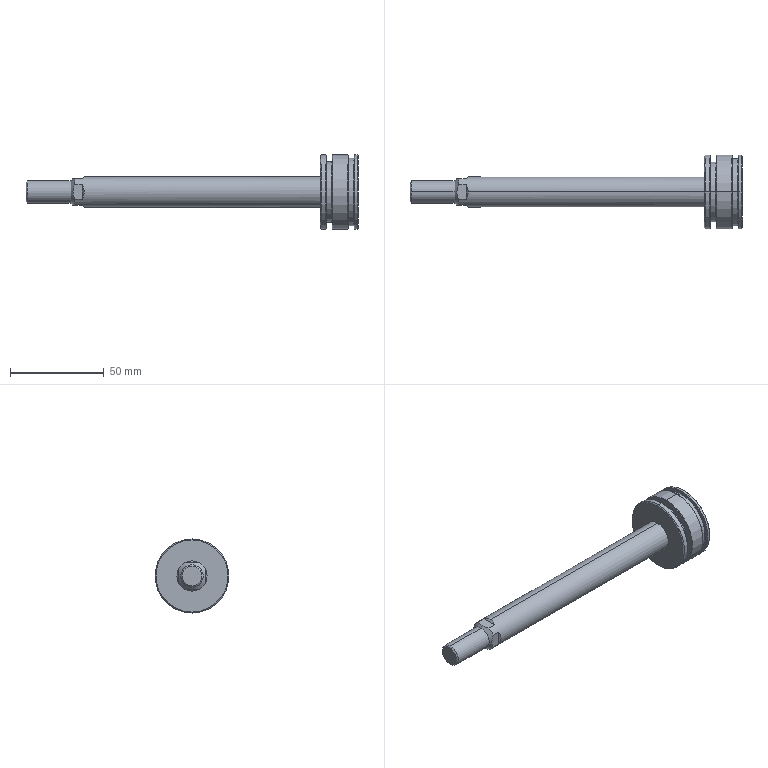Component | SolidWorks | MAL_40x75_S_U_r-1 | 1 solid | 53 faces | box 177 x 39.5 x 39.5 mm | volume 51691 mm3 | cone 16 | plane 15 | cylinder 14 | torus 8 | commonest cylinder face diameters 39.5 x6 12 x2 16 x2 32 x2 36 x2
build123d program:
from build123d import *

# Parameters (mm, degrees)
EXTRUDE1_DEPTH      = 8
EXTRUDE1_DEPTH_BACK = 8
EXTRUDE2_DEPTH      = 8
EXTRUDE2_DEPTH_BACK = 8


with BuildPart() as part:
    # Sketch1 → Revolve1 (revolve)
    with BuildSketch(Plane.XY, mode=Mode.PRIVATE) as revolve1_sk:
        with BuildLine():
            Line((-46, 0), (-46, 5.233))
            Line((-46, 5.233), (-45.233, 6))
            Line((-45.233, 6), (-22, 6))
            Line((-22, 6), (-20, 8))
            Line((-20, 8), (111, 8))
            Line((111, 8), (111, 19.25))
            Line((111, 19.25), (111.5, 19.75))
            Line((111.5, 19.75), (113.9, 19.75))
            Line((113.9, 19.75), (114.1, 19.55))
            Line((114.1, 19.55), (114.1, 16.2))
            ThreePointArc((114.1, 16.2), (114.159, 16.059), (114.3, 16))
            Line((114.3, 16), (117.1, 16))
            ThreePointArc((117.1, 16), (117.241, 16.059), (117.3, 16.2))
            Line((117.3, 16.2), (117.3, 19.55))
            Line((117.3, 19.55), (117.5, 19.75))
            Line((117.5, 19.75), (125.5, 19.75))
            Line((125.5, 19.75), (125.7, 19.55))
            Line((125.7, 19.55), (125.7, 18.2))
            ThreePointArc((125.7, 18.2), (125.759, 18.059), (125.9, 18))
            Line((125.9, 18), (128.8, 18))
            ThreePointArc((128.8, 18), (128.941, 18.059), (129, 18.2))
            Line((129, 18.2), (129, 19.55))
            Line((129, 19.55), (129.2, 19.75))
            Line((129.2, 19.75), (130.5, 19.75))
            Line((130.5, 19.75), (131, 19.25))
            Line((131, 19.25), (131, 0))
            Line((131, 0), (-46, 0))
        make_face()
    revolve(revolve1_sk.sketch.rotate(Axis((131, 0, 0), (-1, 0, 0)), 270), axis=Axis((131, 0, 0), (-1, 0, 0)))

    # Sketch2 → Extrude1 (cut, two sides: drawn at the far end of the back side and taken through both)
    with BuildSketch(Plane(origin=(0, 0, 0), x_dir=(1, 0, 0), z_dir=(0, 1, 0)).offset(-EXTRUDE1_DEPTH_BACK)):
        Polygon((-60, 14), (-60, -14), (-15, -14), (-15, -8), (-16, -7), (-47, -7), (-47, 7), (-16, 7), (-15, 8), (-15, 14), align=None)
    extrude(amount=EXTRUDE1_DEPTH + EXTRUDE1_DEPTH_BACK, mode=Mode.SUBTRACT)

    # Sketch3 → Extrude2 (cut, two sides: drawn at the far end of the back side and taken through both)
    with BuildSketch(Plane.XY.offset(-EXTRUDE2_DEPTH_BACK)):
        Polygon((-60, 14), (-60, -14), (-15, -14), (-15, -8), (-16, -7), (-47, -7), (-47, 7), (-16, 7), (-15, 8), (-15, 14), align=None)
    extrude(amount=EXTRUDE2_DEPTH + EXTRUDE2_DEPTH_BACK, mode=Mode.SUBTRACT)


solid = part.part

# Placed as in the assembly
solid = solid.moved(Location((-15.25, 0, 0), (0, 0, 0)))